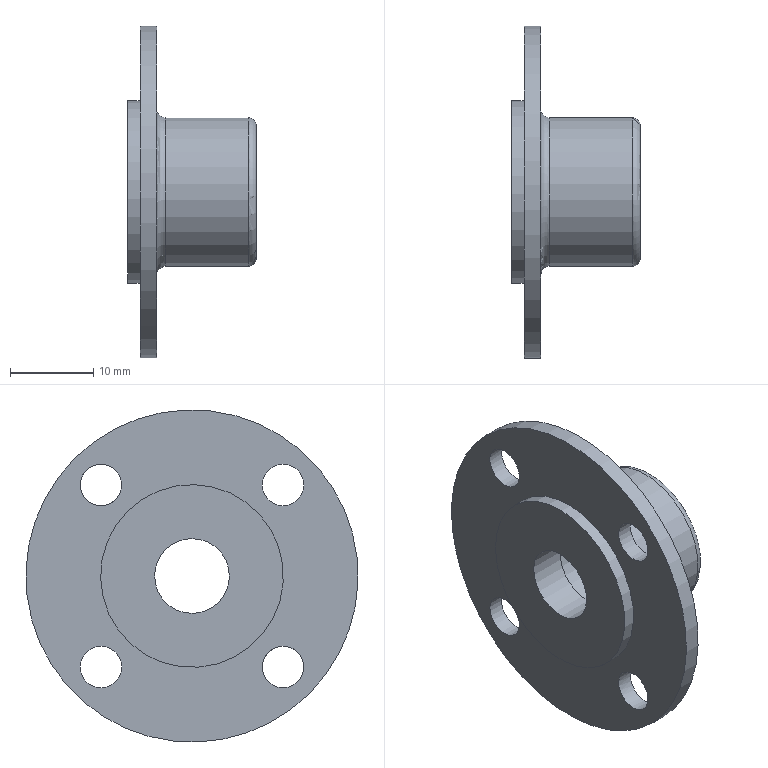Component | NX | LOWER_END_CAP | 1 solid | 16 faces | volume 4830 mm3 | cylinder 9 | plane 5 | torus 2 | commonest cylinder face diameters 5 x4 18 x1 40 x1 22 x1 10 x1 9 x1